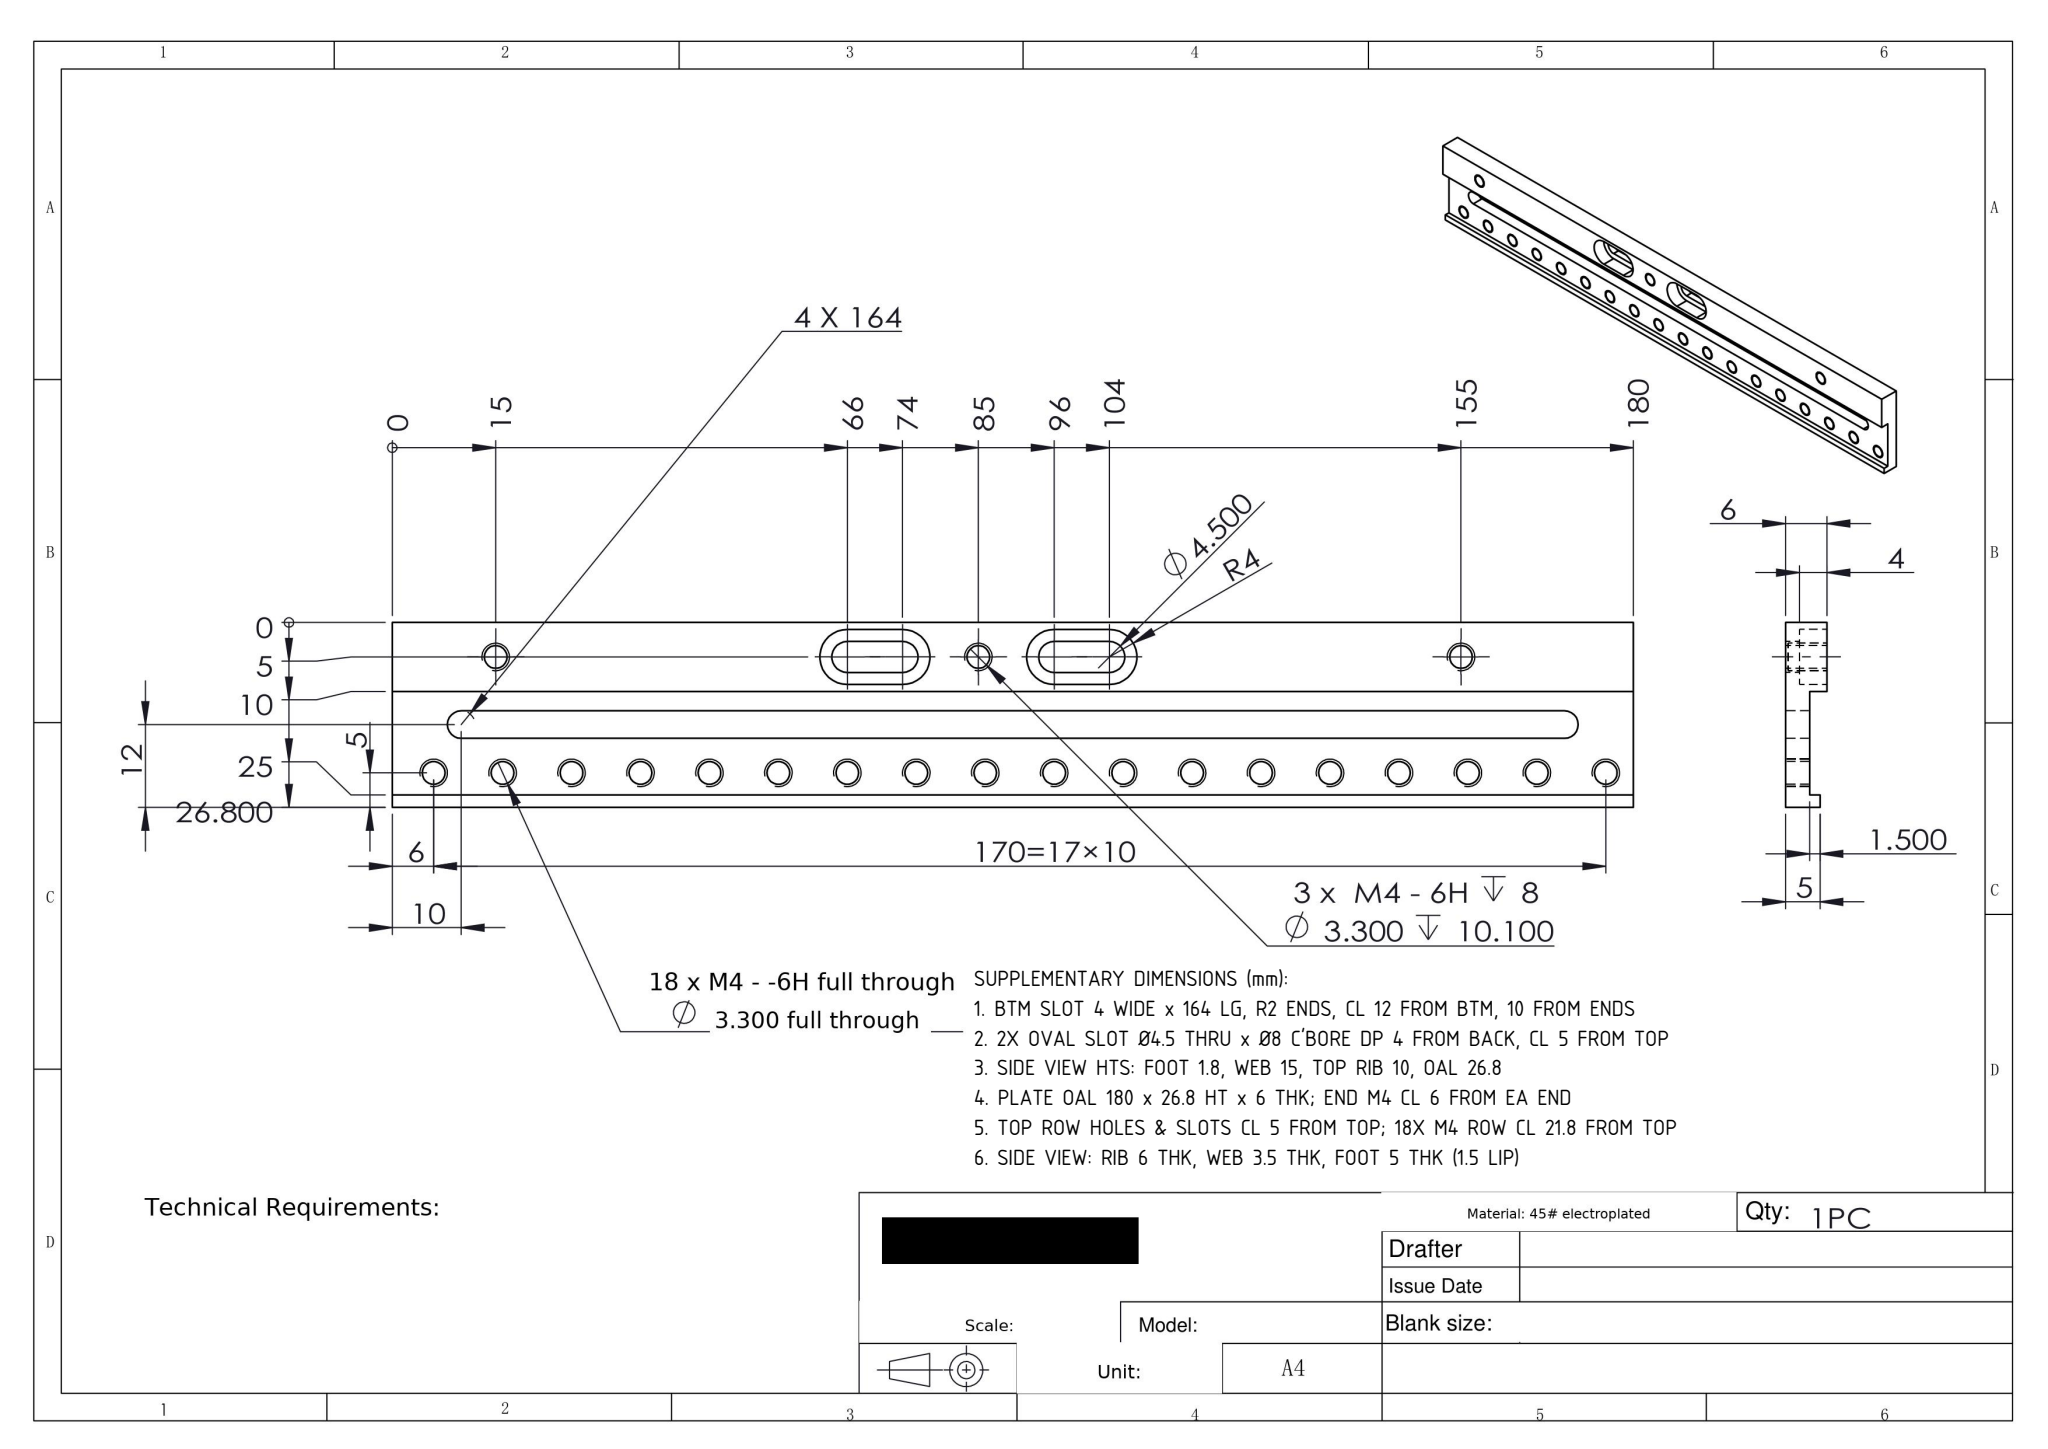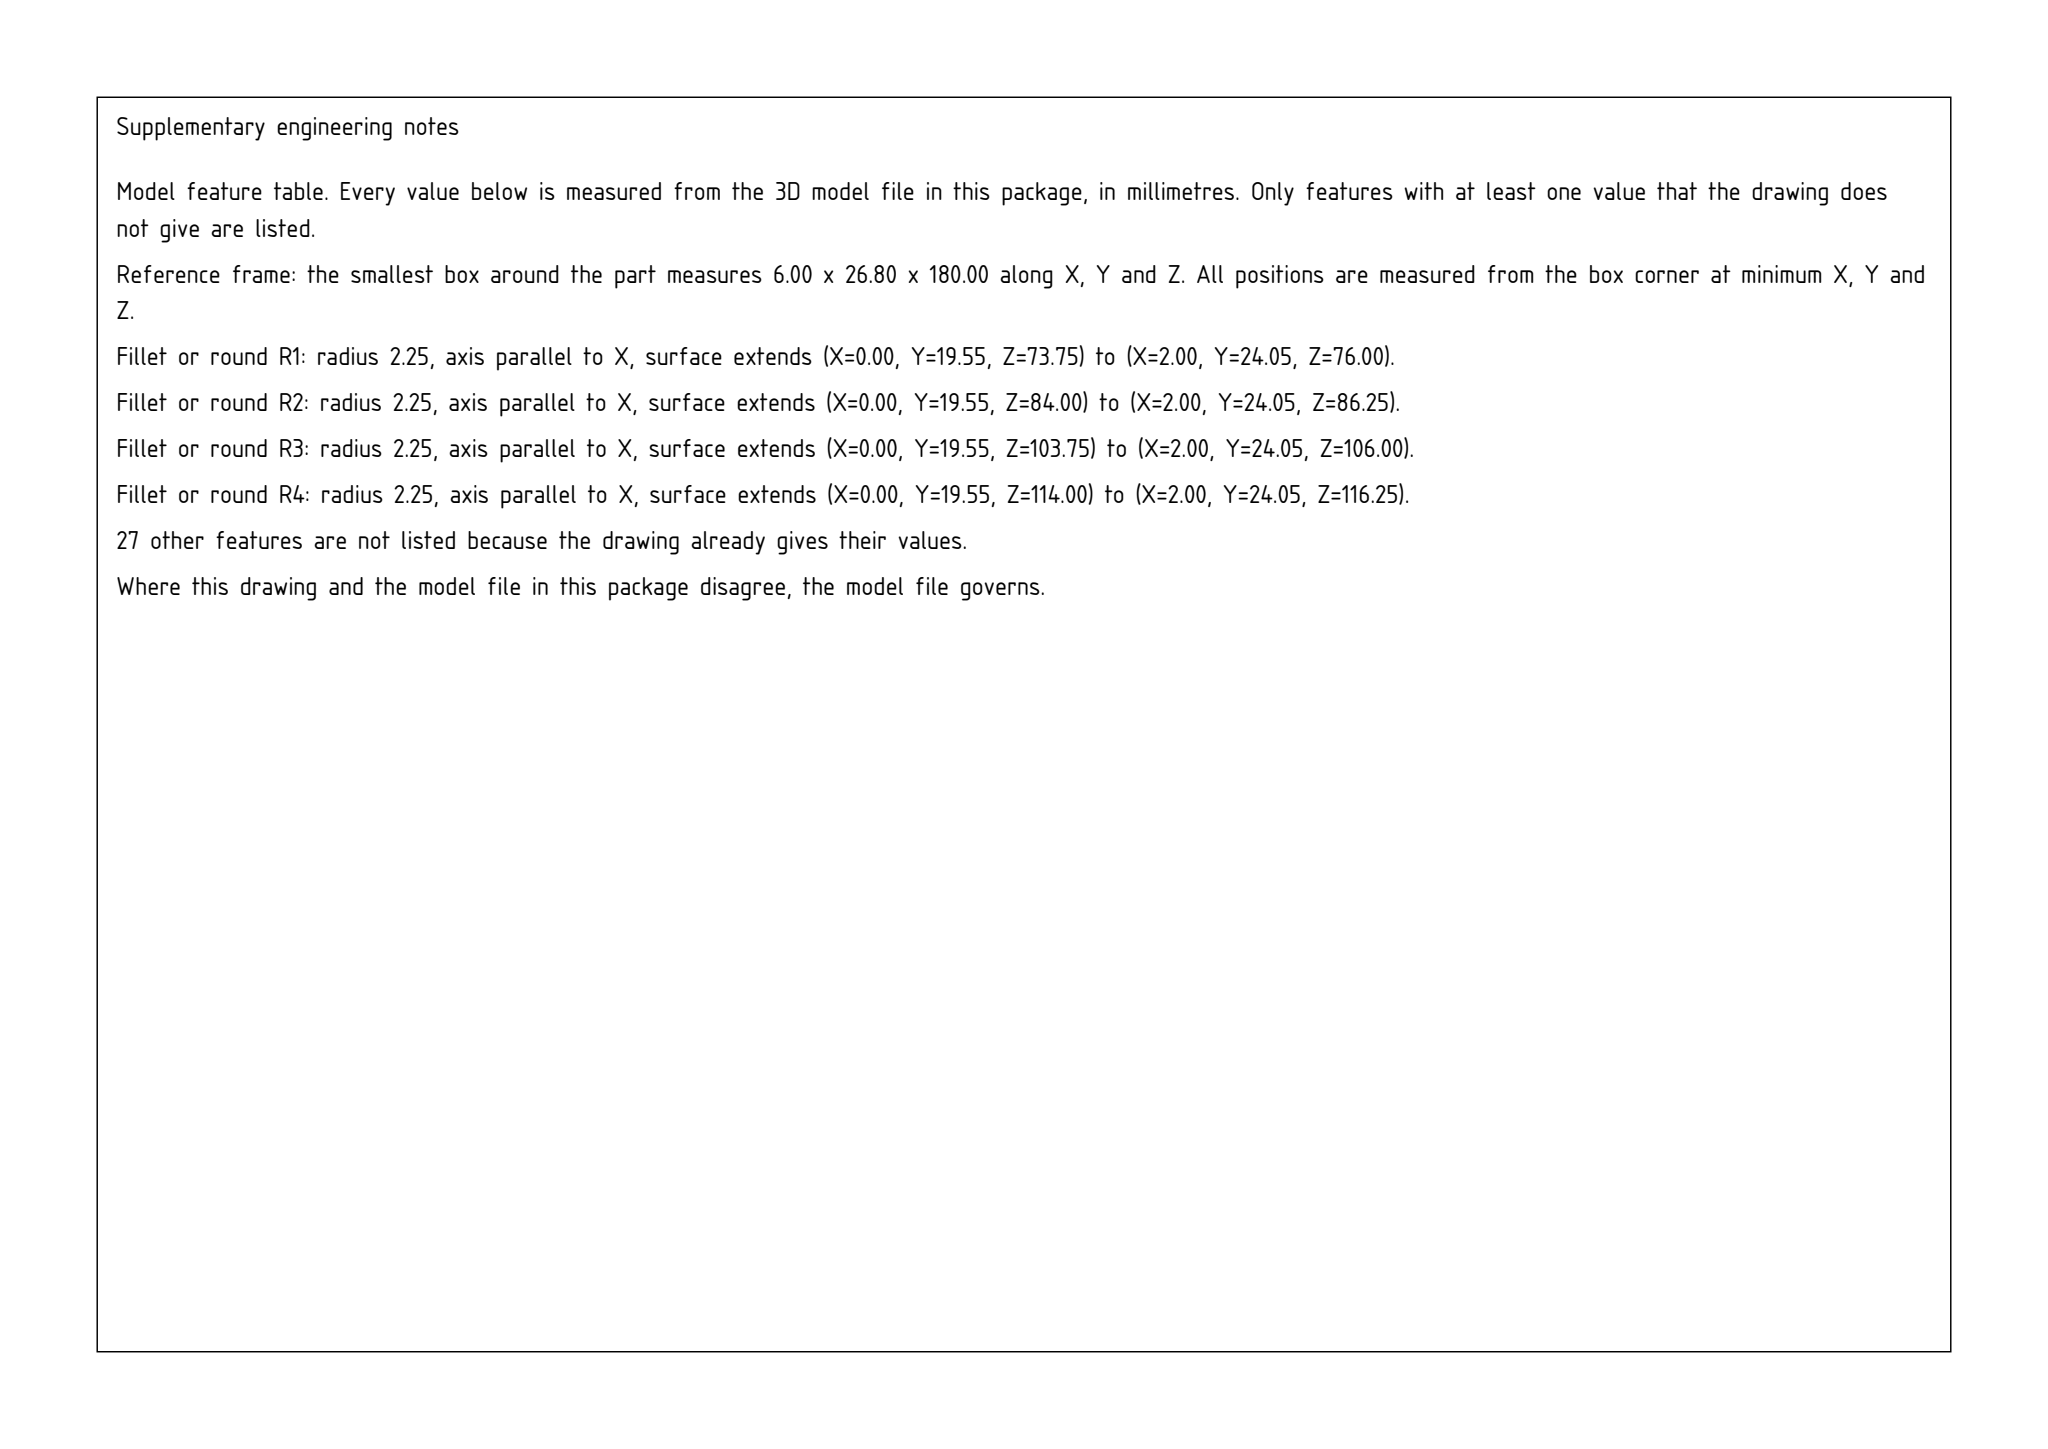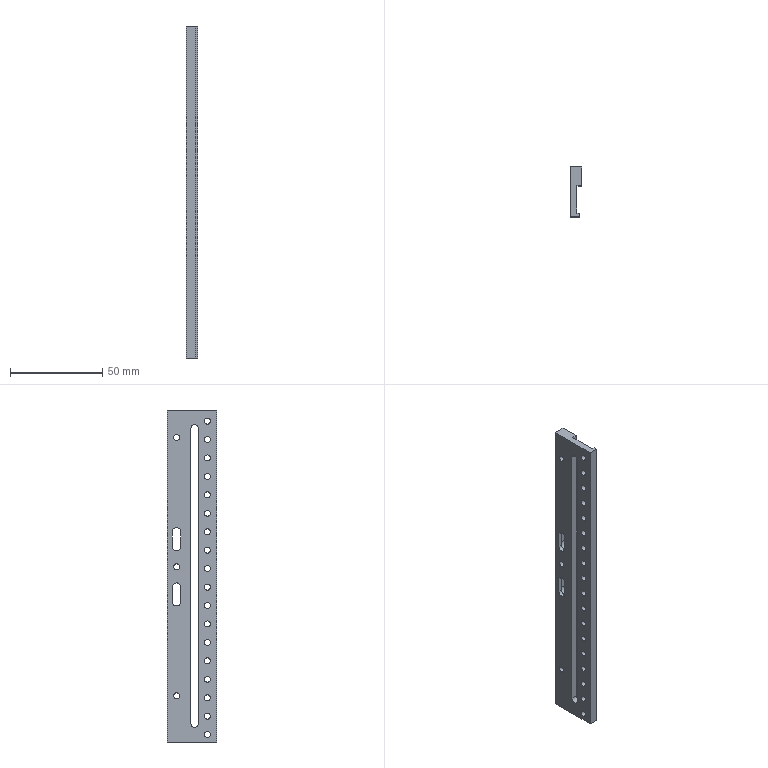Part | SolidWorks | mm | 1 solid | 76 faces | box 6 x 26.8 x 180 mm | volume 17771 mm3 | cylinder 54 | plane 22 | commonest cylinder face diameters 3.3 x42 4.5 x6 8 x4 4 x2
build123d program:
from build123d import *

# Parameters (mm, degrees)
EXTRUDE1_DEPTH                                  = 180
M4_HEX_SOCKET_HEAD_CAP_SCREW_CBORE1_D           = 4.5
M4_HEX_SOCKET_HEAD_CAP_SCREW_CBORE1_CBORE_D     = 8
M4_HEX_SOCKET_HEAD_CAP_SCREW_CBORE1_CBORE_DEPTH = 4
M4_TAPPED_HOLE1_D                               = 3.3
M4_TAPPED_HOLE1_DEPTH                           = 10.1
M4_TAPPED_HOLE1_TIP                             = 0.9914
CUT_EXTRUDE1_DEPTH                              = 4
CUT_EXTRUDE2_DEPTH                              = 10
M4_TAPPED_HOLE2_D                               = 3.3
CUT_EXTRUDE3_DEPTH                              = 183.018


with BuildPart() as part:
    # Sketch1 → Extrude1 (new body)
    with BuildSketch(Plane.XY):
        Polygon((0, 0), (0, 26.8), (6, 26.8), (6, 16.8), (3.5, 16.8), (3.5, 1.8), (5, 1.8), (5, 0), align=None)
    extrude(amount=EXTRUDE1_DEPTH)

    # M4 Hex Socket Head Cap Screw CBORE1 (through all)
    with Locations(Plane(origin=(6, 0, 0), x_dir=(0, 0, -1), z_dir=(1, 0, 0))):
        with Locations((-110, 21.8), (-80, 21.8)):
            CounterBoreHole(M4_HEX_SOCKET_HEAD_CAP_SCREW_CBORE1_D / 2, M4_HEX_SOCKET_HEAD_CAP_SCREW_CBORE1_CBORE_D / 2, M4_HEX_SOCKET_HEAD_CAP_SCREW_CBORE1_CBORE_DEPTH)

    # M4 Tapped Hole1
    with Locations(Plane(origin=(6, 0, 0), x_dir=(0, 0, -1), z_dir=(1, 0, 0))):
        with Locations((-25, 21.8), (-95, 21.8), (-165, 21.8)):
            Hole(M4_TAPPED_HOLE1_D / 2, depth=M4_TAPPED_HOLE1_DEPTH)
            with Locations((0, 0, -(M4_TAPPED_HOLE1_DEPTH + M4_TAPPED_HOLE1_TIP / 2))):  # 118° drill point
                Cone(0, M4_TAPPED_HOLE1_D / 2, M4_TAPPED_HOLE1_TIP, mode=Mode.SUBTRACT)

    # Sketch6 → Cut-Extrude1 (cut)
    with BuildSketch(Plane(origin=(6, 0, 0), x_dir=(0, 0, -1), z_dir=(1, 0, 0))):
        with BuildLine():
            Line((-84, 25.8), (-76, 25.8))
            ThreePointArc((-76, 25.8), (-72, 21.8), (-76, 17.8))
            Line((-76, 17.8), (-84, 17.8))
            ThreePointArc((-84, 17.8), (-88, 21.8), (-84, 25.8))
        make_face()
        with BuildLine():
            Line((-114, 25.8), (-106, 25.8))
            ThreePointArc((-106, 25.8), (-102, 21.8), (-106, 17.8))
            Line((-106, 17.8), (-114, 17.8))
            ThreePointArc((-114, 17.8), (-118, 21.8), (-114, 25.8))
        make_face()
    extrude(amount=-CUT_EXTRUDE1_DEPTH, mode=Mode.SUBTRACT)

    # Sketch7 → Cut-Extrude2 (cut)
    with BuildSketch(Plane(origin=(2, 0, 0), x_dir=(0, 0, -1), z_dir=(1, 0, 0))):
        with BuildLine():
            Line((-114, 24.05), (-106, 24.05))
            ThreePointArc((-106, 24.05), (-103.75, 21.8), (-106, 19.55))
            Line((-106, 19.55), (-114, 19.55))
            ThreePointArc((-114, 19.55), (-116.25, 21.8), (-114, 24.05))
        make_face()
        with BuildLine():
            Line((-84, 24.05), (-76, 24.05))
            ThreePointArc((-76, 24.05), (-73.75, 21.8), (-76, 19.55))
            Line((-76, 19.55), (-84, 19.55))
            ThreePointArc((-84, 19.55), (-86.25, 21.8), (-84, 24.05))
        make_face()
    extrude(amount=-CUT_EXTRUDE2_DEPTH, mode=Mode.SUBTRACT)

    # M4 Tapped Hole2 (through all)
    with Locations(Plane(origin=(3.5, 0, 0), x_dir=(0, 0, -1), z_dir=(1, 0, 0))):
        with Locations((-174, 5), (-164, 5), (-154, 5), (-144, 5), (-134, 5), (-124, 5), (-114, 5), (-104, 5), (-94, 5), (-84, 5), (-74, 5), (-64, 5), (-54, 5), (-44, 5), (-34, 5), (-24, 5), (-14, 5), (-4, 5)):
            Hole(M4_TAPPED_HOLE2_D / 2)

    # Sketch11 → Cut-Extrude3 (cut, through all)
    with BuildSketch(Plane(origin=(3.5, 0, 0), x_dir=(0, 0, -1), z_dir=(1, 0, 0))):
        with BuildLine():
            Line((-170, 14), (-10, 14))
            ThreePointArc((-10, 14), (-8, 12), (-10, 10))
            Line((-10, 10), (-170, 10))
            ThreePointArc((-170, 10), (-172, 12), (-170, 14))
        make_face()
    extrude(amount=-CUT_EXTRUDE3_DEPTH, mode=Mode.SUBTRACT)


solid = part.part